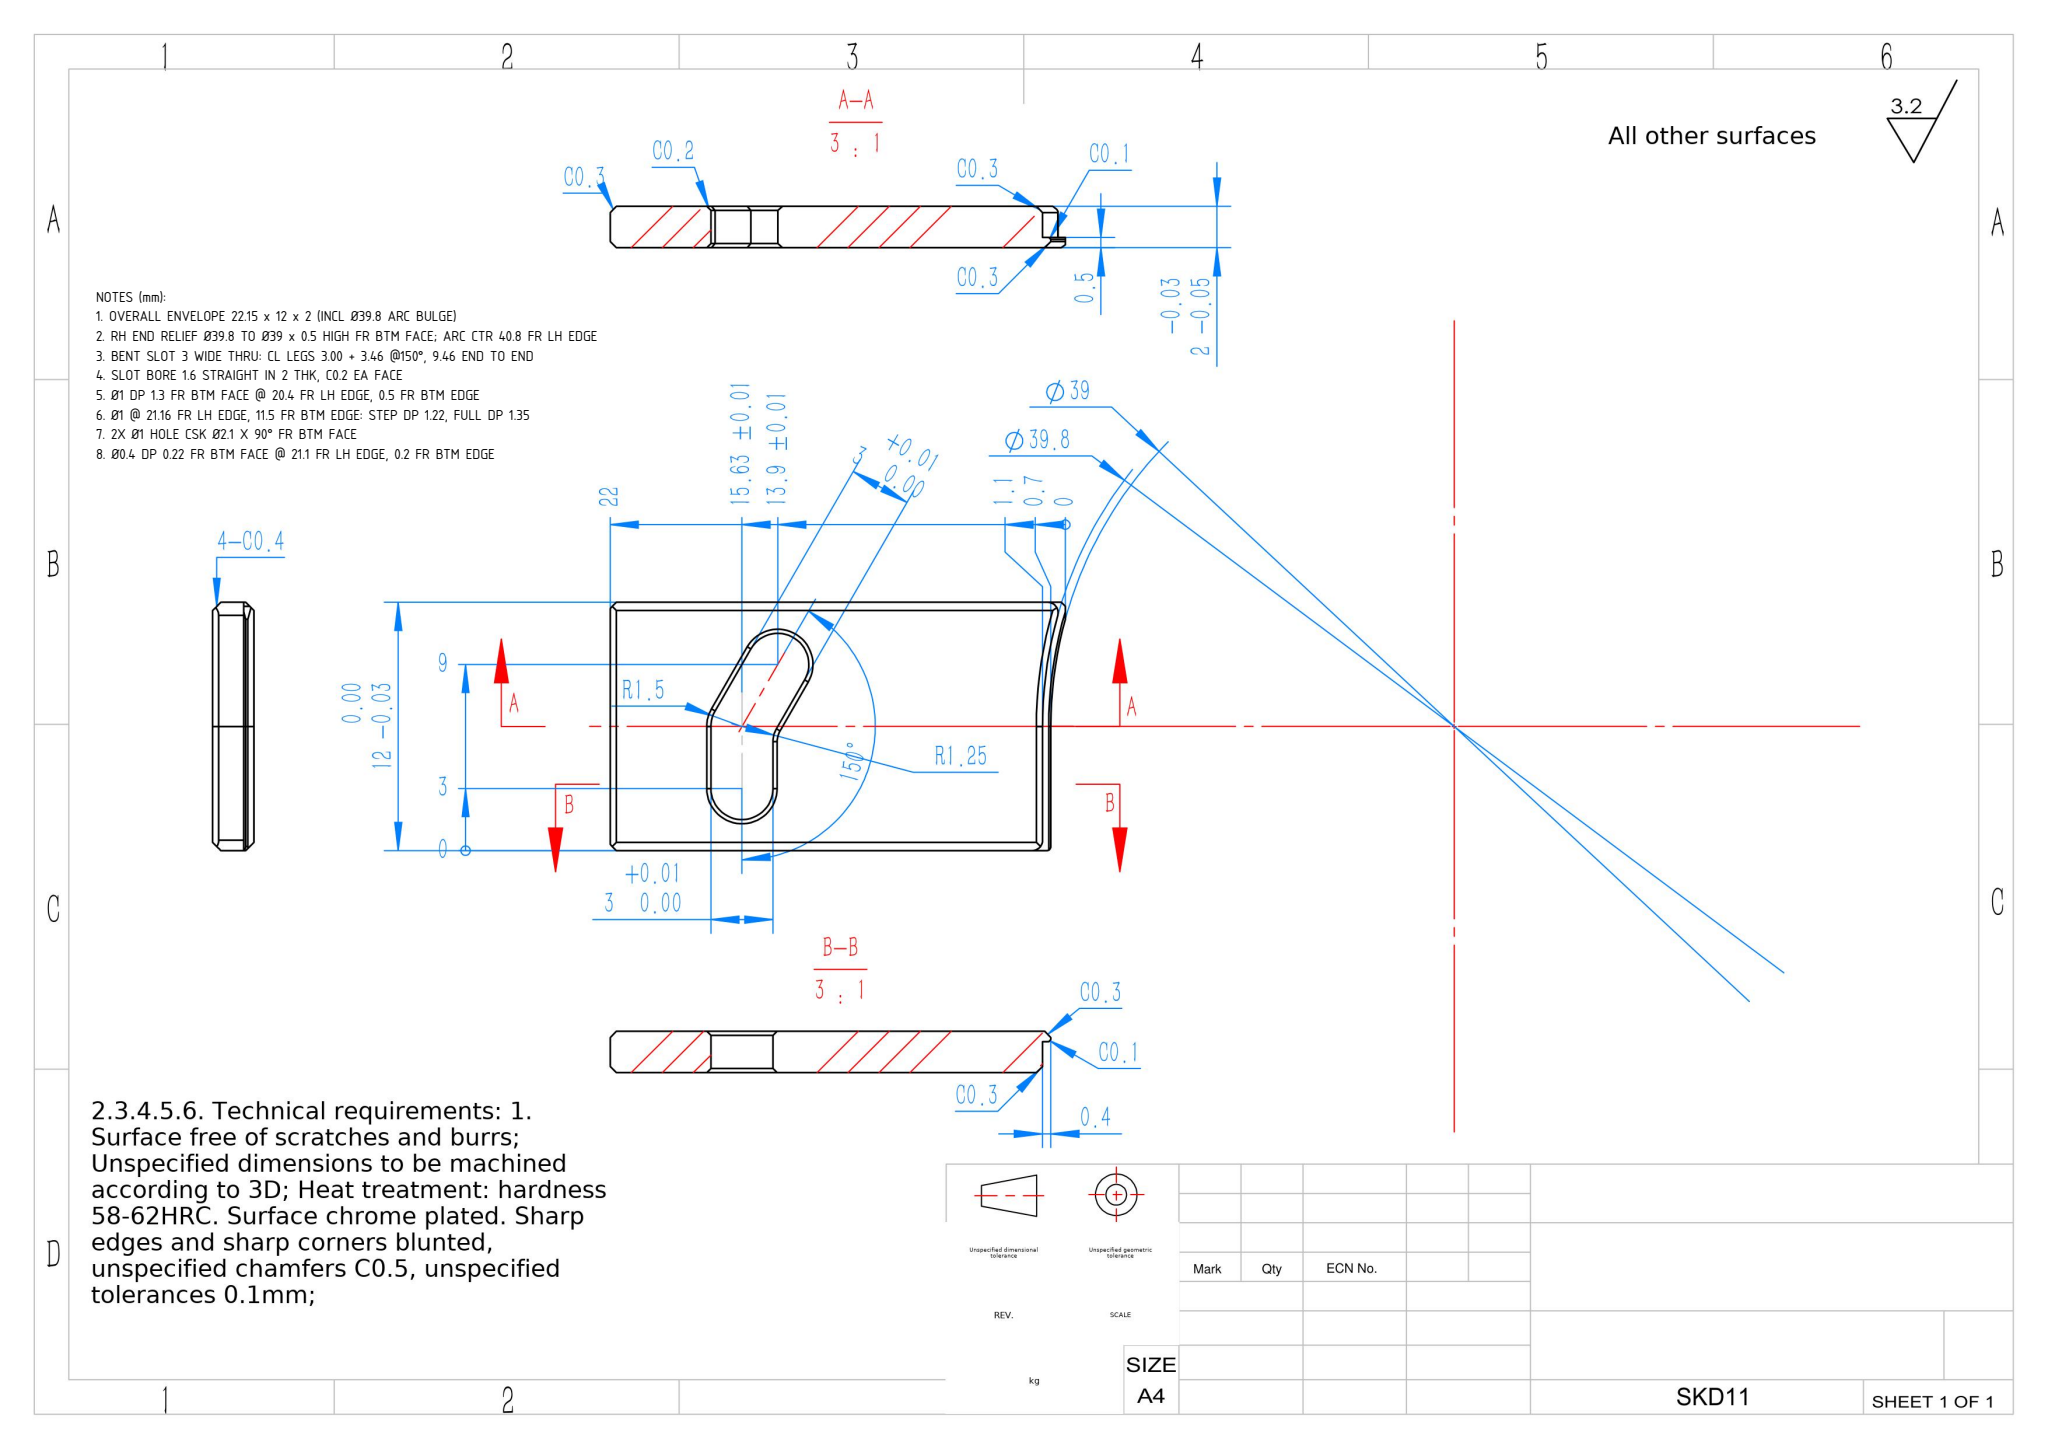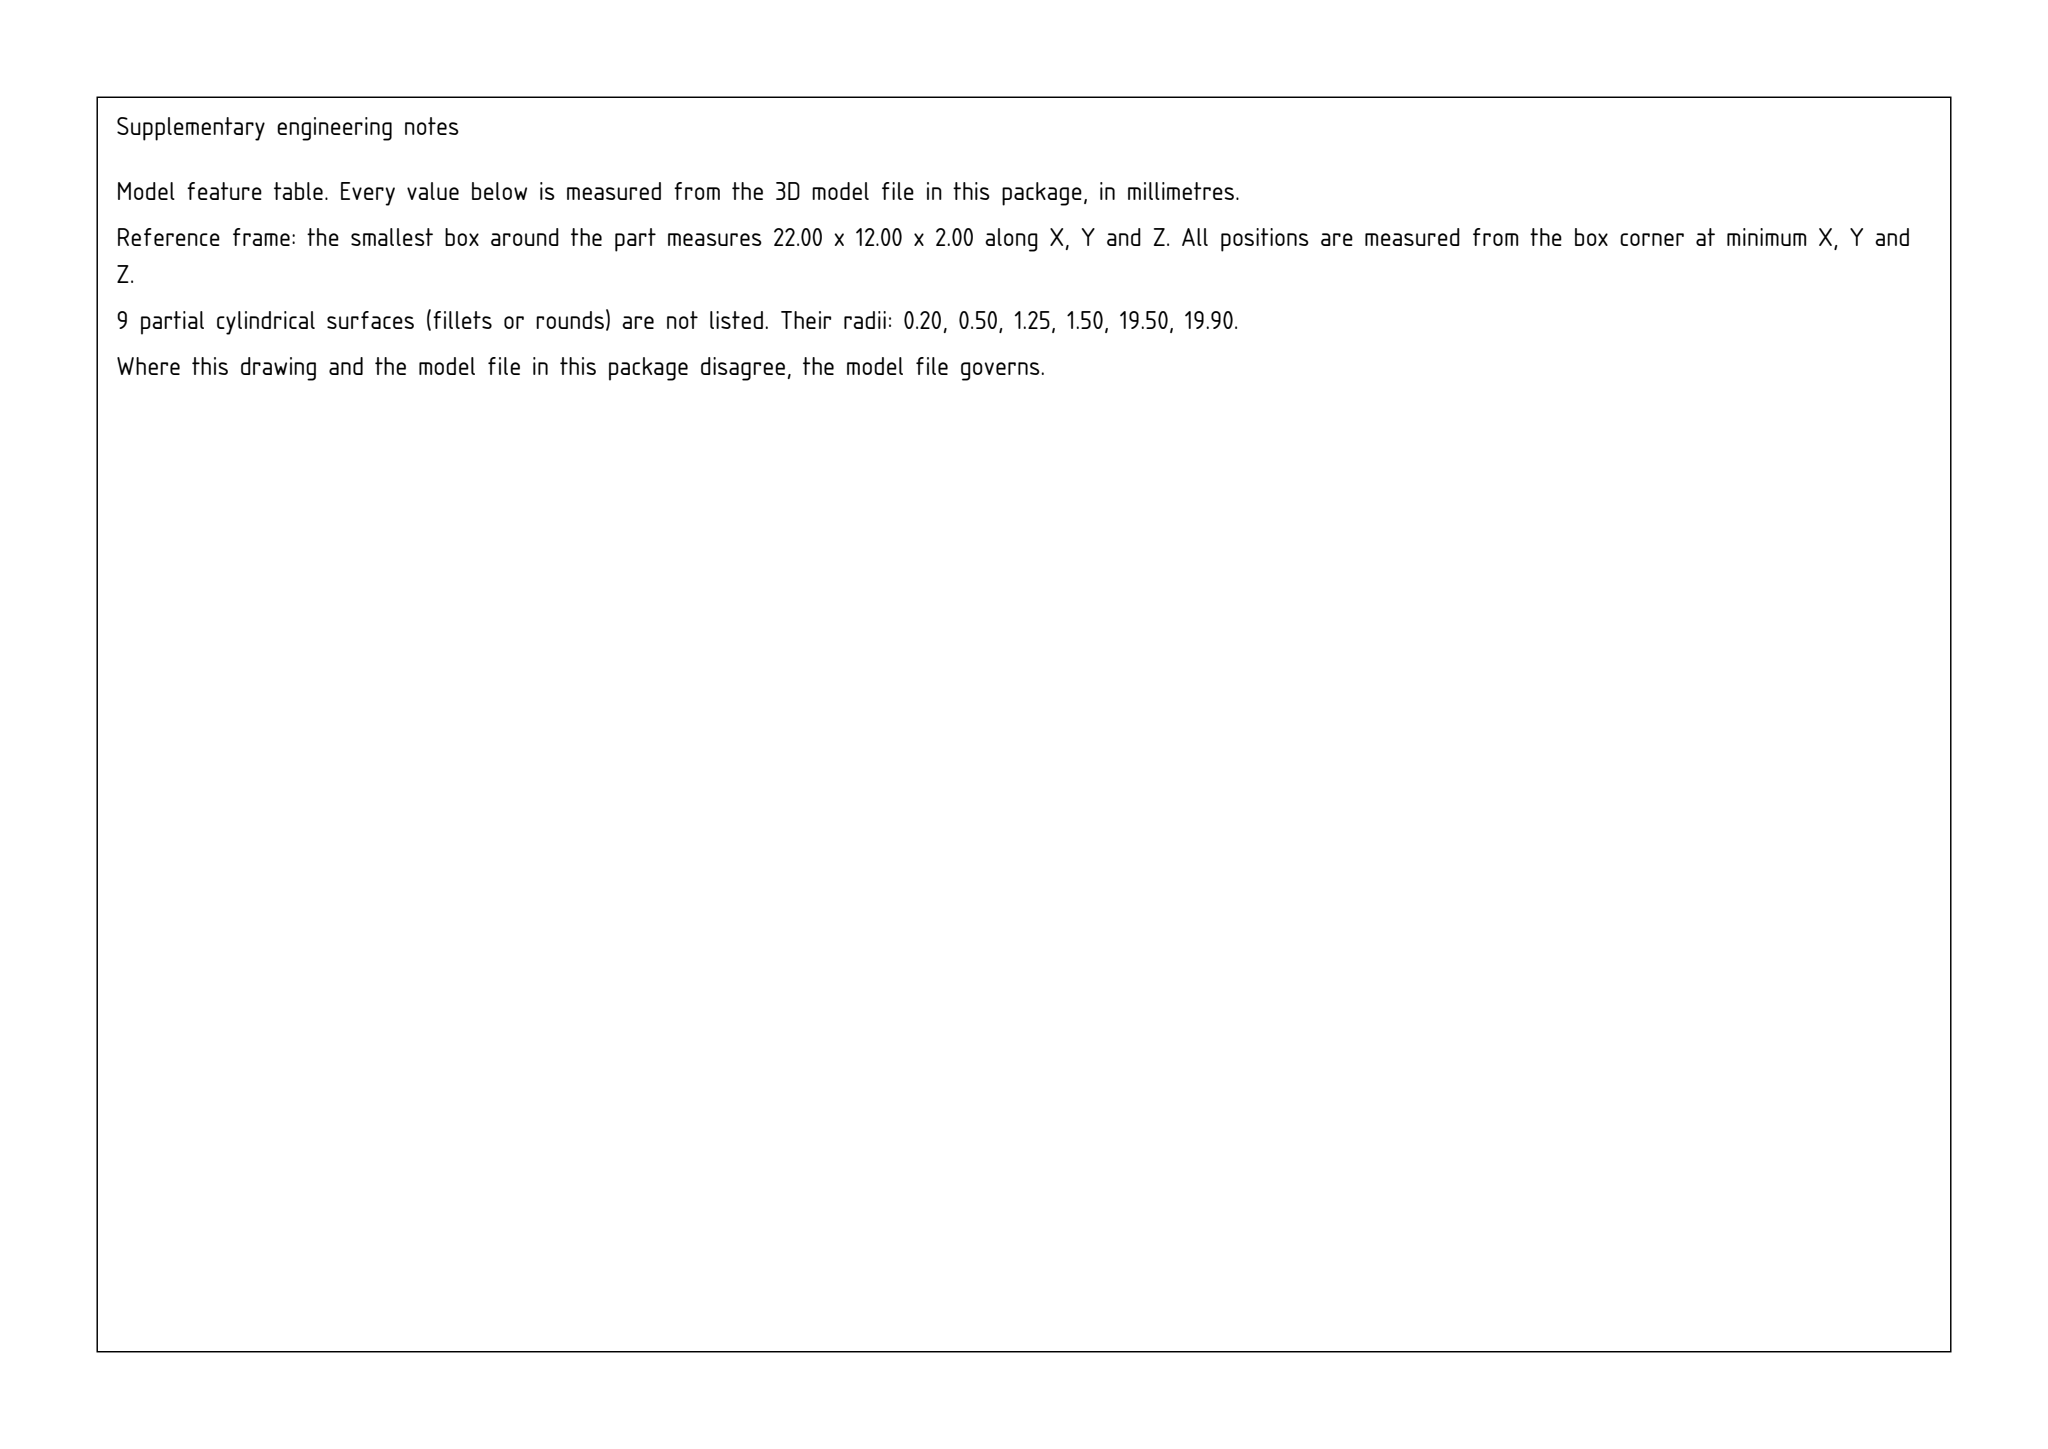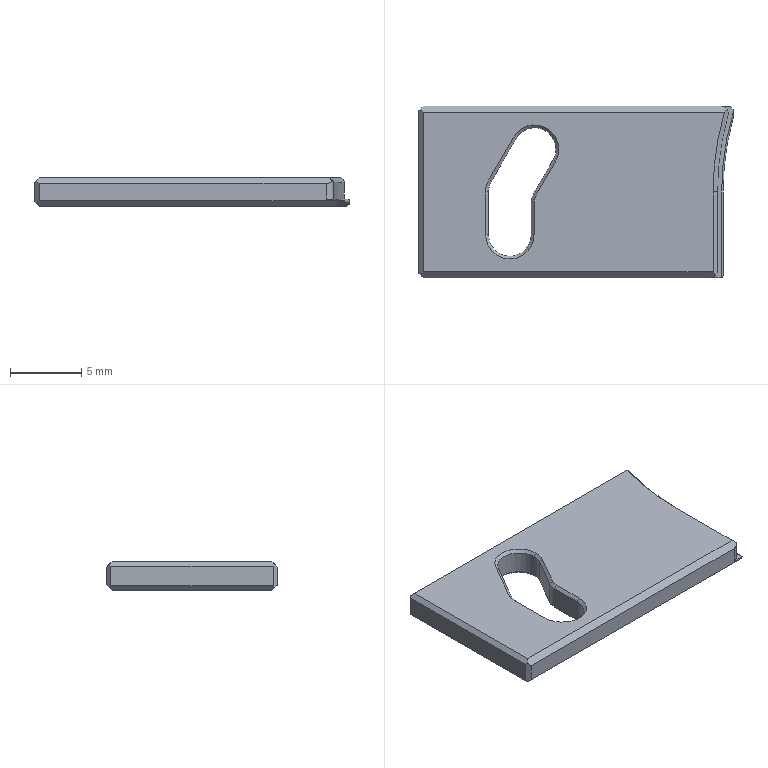Part | SolidWorks | mm | 1 solid | 56 faces | box 22 x 12 x 2 mm | volume 445 mm3 | plane 33 | cone 12 | cylinder 11 | commonest cylinder face diameters 3 x4 1 x3 39.8 x1 39 x1 2.5 x1 0.4 x1
Drawing notes:
OVERALL ENVELOPE 22.15 x 12 x 2 (INCL Ø39.8 ARC BULGE) | from the solid: bbox_xyz 22.151 x 12.0 x 2.0; z-planes 0 and 2.0
RH END RELIEF Ø39.8 TO Ø39 x 0.5 HIGH FR BTM FACE; ARC CTR 40.8 FR LH EDGE | from the solid: x-planes 20.9 & 21.3 (0.4 apart) = Ø39.8 r19.9 / Ø39 r19.5 about ctr x=40.8, y=6.0; z-planes 0 & 0.5
BENT SLOT 3 WIDE THRU: CL LEGS 3.00 + 3.46 @150°, 9.46 END TO END | from the solid: R1.5 end ctrs (6.37,3.0) & (8.1,9.0), bend ctr (6.37,6.0): leg1=3.00, leg2=3.46, +2xR1.5=9.46; R1.25 fillet ctr (9.12,5.26)
SLOT BORE 1.6 STRAIGHT IN 2 THK, C0.2 EA FACE | from the solid: Ø3.0 cyls len 1.6; 90° cones ref Ø3.0/Ø3.4 = 0.2 chamfer each face; 1.6+0.2+0.2=2.0
Ø1 DP 1.3 FR BTM FACE @ 20.4 FR LH EDGE, 0.5 FR BTM EDGE | from the solid: cyl Ø1.0 axis z at (20.4,0.5), length 1.3 of 2.0 thk
Ø1 @ 21.16 FR LH EDGE, 11.5 FR BTM EDGE: STEP DP 1.22, FULL DP 1.35 | from the solid: coaxial Ø1.0 z-cyls at (21.16,11.5), lengths 1.22 and 1.35 from z=0
2X Ø1 HOLE CSK Ø2.1 X 90° FR BTM FACE | from the solid: cones[90.0,2.1] count 2 on the Ø1 holes at (20.4,0.5) and (21.16,11.5)
Ø0.4 DP 0.22 FR BTM FACE @ 21.1 FR LH EDGE, 0.2 FR BTM EDGE | from the solid: cyl Ø0.4 axis z at (21.1,0.2), length 0.22 of 2.0 thk